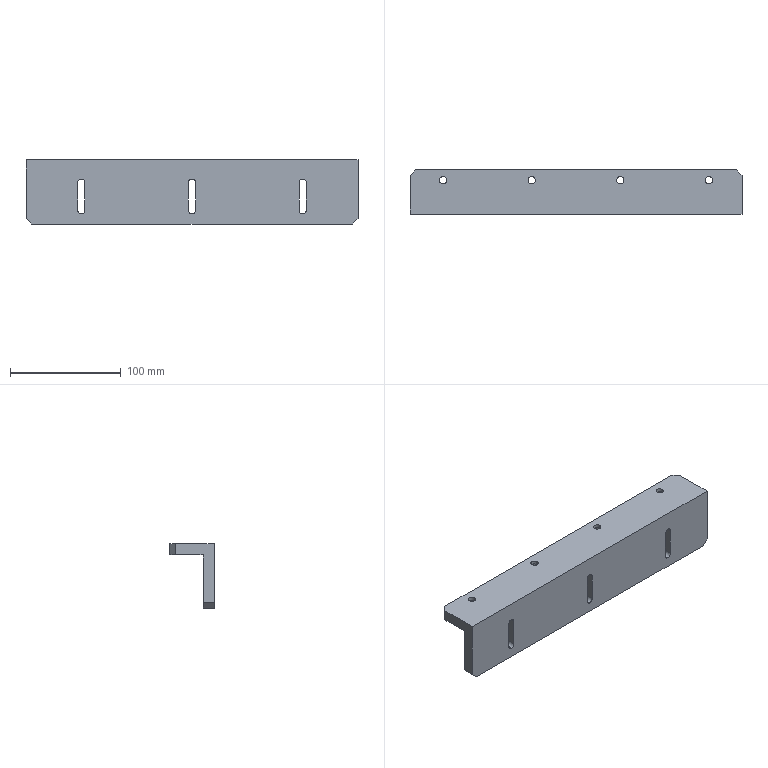Component | SolidWorks | P-SLJ-001-006-3 | 1 solid | 47 faces | box 300 x 40 x 58 mm | volume 254607 mm3 | cylinder 25 | plane 22 | commonest cylinder face diameters 6.5 x9 11 x8 6.6 x8 | material 45#
build123d program:
from build123d import *

# Parameters (mm, degrees)
EXTRUDE1_DEPTH                                       = 150
CBORE_FOR_M6_HEXAGON_SOCKET_HEAD_CAP_SCR_D           = 6.6
CBORE_FOR_M6_HEXAGON_SOCKET_HEAD_CAP_SCR_CBORE_D     = 11
CBORE_FOR_M6_HEXAGON_SOCKET_HEAD_CAP_SCR_CBORE_DEPTH = 6.8
EXTRUDE2_DEPTH                                       = 164.597
CHAMFER1_SIZE                                        = 5


with BuildPart() as part:
    # Sketch1 → Extrude1 (new, symmetric)
    with BuildSketch(Plane(origin=(0, 0, 0), x_dir=(0, 0, -1), z_dir=(1, 0, 0))):
        Polygon((0, 0), (-58, 0), (-58, 10), (-10, 10), (-10, 40), (0, 40), align=None)
    extrude(amount=EXTRUDE1_DEPTH, both=True)

    # CBORE for M6 Hexagon socket head cap scr (through all)
    with Locations(Plane.XY.offset(10)):
        with Locations((-120, 30.5), (-40, 30.5), (40, 30.5), (120, 30.5)):
            CounterBoreHole(CBORE_FOR_M6_HEXAGON_SOCKET_HEAD_CAP_SCR_D / 2, CBORE_FOR_M6_HEXAGON_SOCKET_HEAD_CAP_SCR_CBORE_D / 2, CBORE_FOR_M6_HEXAGON_SOCKET_HEAD_CAP_SCR_CBORE_DEPTH)

    # Sketch4 → Extrude2 (cut, through all)
    with BuildSketch(Plane(origin=(0, 10, 0), x_dir=(1, 0, 0), z_dir=(0, 1, 0))):
        with BuildLine():
            Line((-96.75, -20.5), (-96.75, -45.5))
            ThreePointArc((-96.75, -45.5), (-100, -48.75), (-103.25, -45.5))
            Line((-103.25, -45.5), (-103.25, -20.5))
            ThreePointArc((-103.25, -20.5), (-100, -17.25), (-96.75, -20.5))
        make_face()
        with BuildLine():
            Line((3.25, -20.5), (3.25, -45.5))
            ThreePointArc((3.25, -45.5), (0, -48.75), (-3.25, -45.5))
            Line((-3.25, -45.5), (-3.25, -20.5))
            ThreePointArc((-3.25, -20.5), (0, -17.25), (3.25, -20.5))
        make_face()
        with BuildLine():
            Line((103.25, -20.5), (103.25, -45.5))
            ThreePointArc((103.25, -45.5), (100, -48.75), (96.75, -45.5))
            Line((96.75, -45.5), (96.75, -20.5))
            ThreePointArc((96.75, -20.5), (100, -17.25), (103.25, -20.5))
        make_face()
    extrude(amount=-EXTRUDE2_DEPTH, mode=Mode.SUBTRACT)

    # Chamfer1
    chamfer1_edges = [part.edges().sort_by_distance(p)[0] for p in [
        (150, 5, 58),
        (-150, 5, 58),
        (150, 40, 5),
        (-150, 40, 5),
    ]]
    chamfer(chamfer1_edges, length=CHAMFER1_SIZE)


solid = part.part

# Placed as in the assembly
solid = solid.moved(Location((81.5, -100.5, 991.634), (-180, 0, 180)))